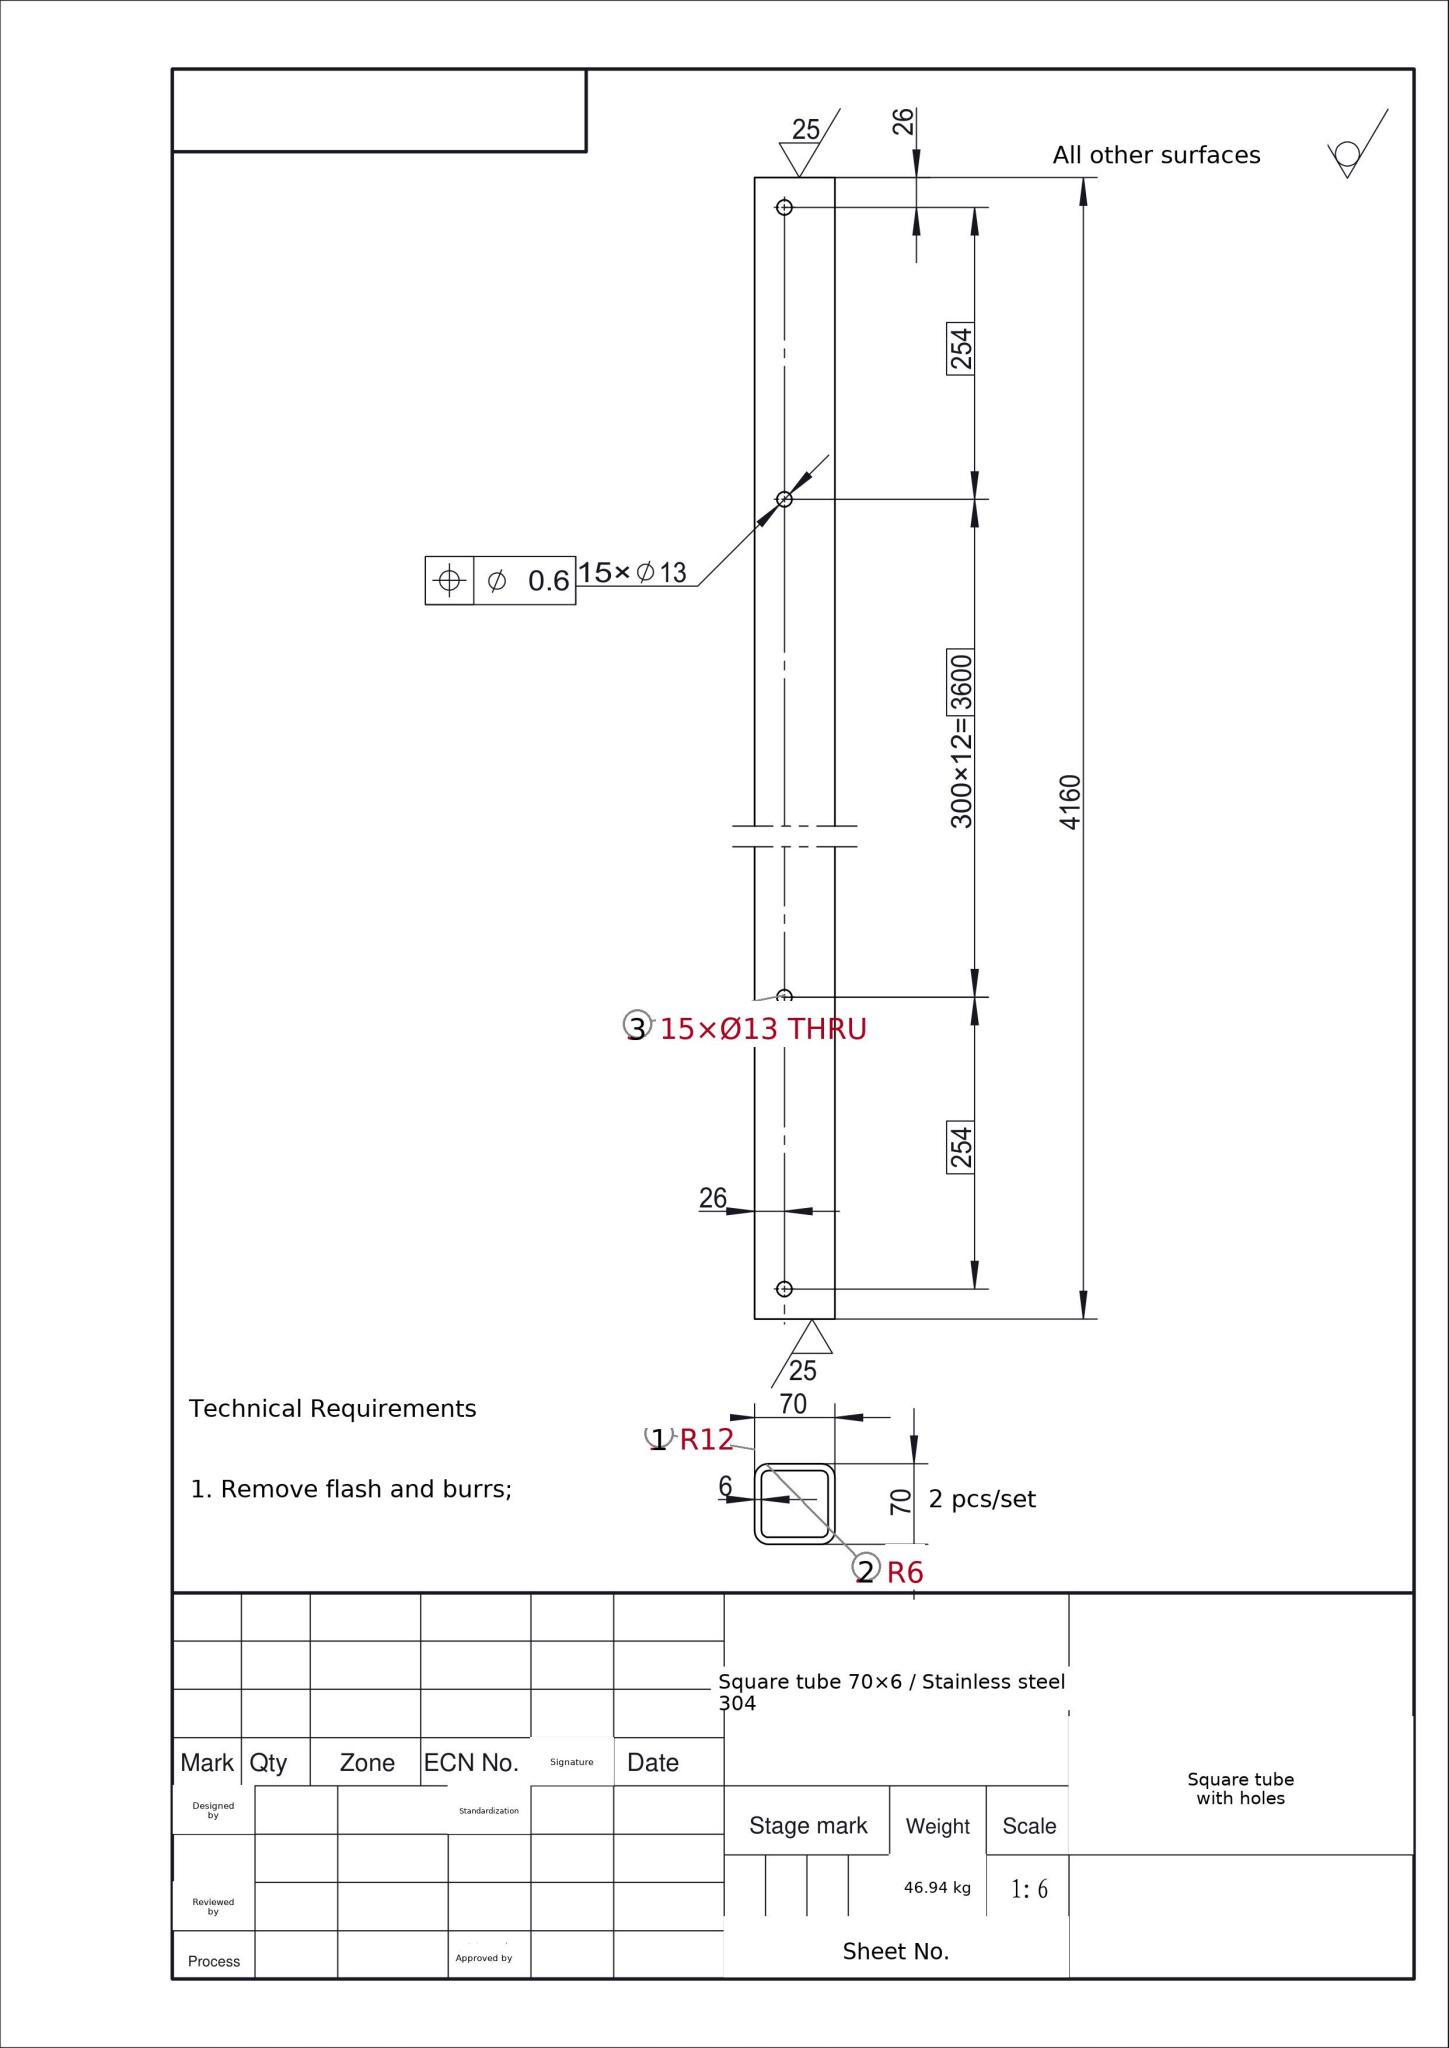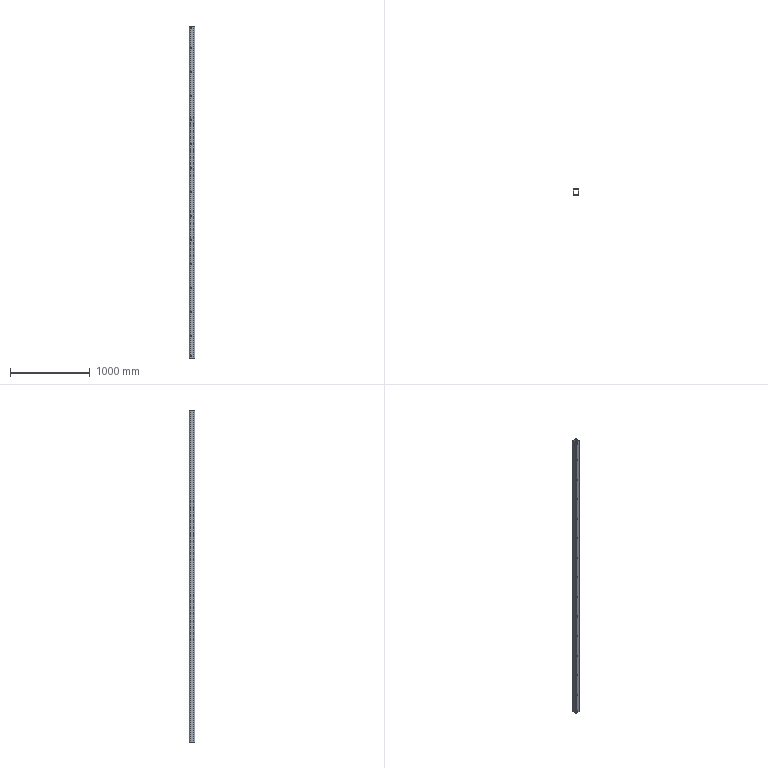Part | SolidWorks | mm | material Square tube 70×6 / Stainless steel 304 | 1 solid | 78 faces | box 70 x 70 x 4160 mm | volume 5980203 mm3 | cylinder 68 | plane 10 | commonest cylinder face diameters 13 x60 24 x4 12 x4
build123d program:
from build123d import *

# Parameters (mm, degrees)
BOSS_EXTRUDE1_DEPTH = 4160
SKETCH2_R           = 6.5
CUT_EXTRUDE1_DEPTH  = 4162.178
SKETCH3_R           = 6.5
CUT_EXTRUDE2_DEPTH  = 4162.178


with BuildPart() as part:
    # Sketch1 → Boss-Extrude1 (new body)
    with BuildSketch(Plane.XY):
        with BuildLine():
            Line((12, 0), (58, 0))
            ThreePointArc((58, 0), (66.485, 3.515), (70, 12))
            Line((70, 12), (70, 58))
            ThreePointArc((70, 58), (66.485, 66.485), (58, 70))
            Line((58, 70), (12, 70))
            ThreePointArc((12, 70), (3.515, 66.485), (0, 58))
            Line((0, 58), (0, 12))
            ThreePointArc((0, 12), (3.515, 3.515), (12, 0))
        make_face()
        with BuildLine():
            Line((12, 6), (58, 6))
            ThreePointArc((58, 6), (62.243, 7.757), (64, 12))
            Line((64, 12), (64, 58))
            ThreePointArc((64, 58), (62.243, 62.243), (58, 64))
            Line((58, 64), (12, 64))
            ThreePointArc((12, 64), (7.757, 62.243), (6, 58))
            Line((6, 58), (6, 12))
            ThreePointArc((6, 12), (7.757, 7.757), (12, 6))
        make_face(mode=Mode.SUBTRACT)
    extrude(amount=BOSS_EXTRUDE1_DEPTH)

    # Sketch2 → Cut-Extrude1 (cut, through all)
    with BuildSketch(Plane(origin=(0, 70, 0), x_dir=(1, 0, 0), z_dir=(0, 1, 0))):
        with Locations(Location((26, -280, 0), (0, 0, 270))):
            Circle(SKETCH2_R)
        with Locations(Location((26, -580, 0), (0, 0, 270))):
            Circle(SKETCH2_R)
        with Locations(Location((26, -880, 0), (0, 0, 270))):
            Circle(SKETCH2_R)
        with Locations(Location((26, -1180, 0), (0, 0, 270))):
            Circle(SKETCH2_R)
        with Locations(Location((26, -1480, 0), (0, 0, 270))):
            Circle(SKETCH2_R)
        with Locations(Location((26, -1780, 0), (0, 0, 270))):
            Circle(SKETCH2_R)
        with Locations(Location((26, -2080, 0), (0, 0, 270))):
            Circle(SKETCH2_R)
        with Locations(Location((26, -2380, 0), (0, 0, 270))):
            Circle(SKETCH2_R)
        with Locations(Location((26, -2680, 0), (0, 0, 270))):
            Circle(SKETCH2_R)
        with Locations(Location((26, -2980, 0), (0, 0, 270))):
            Circle(SKETCH2_R)
        with Locations(Location((26, -3280, 0), (0, 0, 270))):
            Circle(SKETCH2_R)
        with Locations(Location((26, -3580, 0), (0, 0, 270))):
            Circle(SKETCH2_R)
        with Locations(Location((26, -3880, 0), (0, 0, 270))):
            Circle(SKETCH2_R)
    extrude(amount=-CUT_EXTRUDE1_DEPTH, mode=Mode.SUBTRACT)

    # Sketch3 → Cut-Extrude2 (cut, through all)
    with BuildSketch(Plane(origin=(0, 70, 0), x_dir=(1, 0, 0), z_dir=(0, 1, 0))):
        with Locations(Location((26, -26, 0), (0, 0, 270))):
            Circle(SKETCH3_R)
        with Locations(Location((26, -4134, 0), (0, 0, 270))):
            Circle(SKETCH3_R)
    extrude(amount=-CUT_EXTRUDE2_DEPTH, mode=Mode.SUBTRACT)


solid = part.part